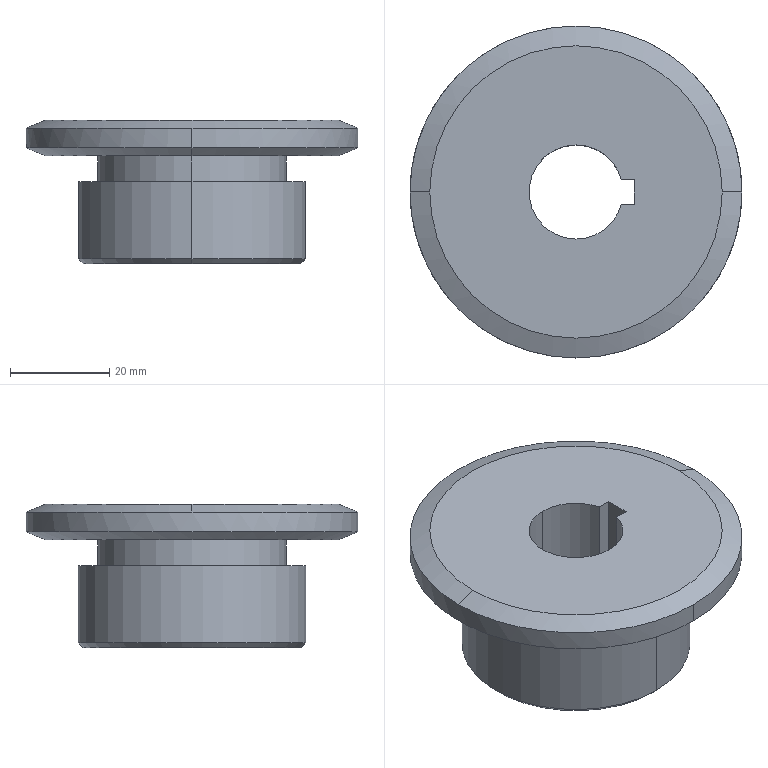Component | SolidWorks | YC1-250-03-01SliderAssembly-1_YC1-200-03-33SmallSprocket-1 | 1 solid | 23 faces | box 67 x 67 x 29 mm | volume 48926 mm3 | cylinder 9 | cone 7 | plane 7 | commonest cylinder face diameters 19 x3 67 x2 46 x2 38 x2 | material Plain Carbon Steel
STEP:
#1=COLOUR_RGB('',0.7922,0.8196,0.9333);
#2=FILL_AREA_STYLE_COLOUR('',#1);
#3=FILL_AREA_STYLE('',(#2));
#4=SURFACE_STYLE_FILL_AREA(#3);
#5=SURFACE_SIDE_STYLE('',(#4));
#6=SURFACE_STYLE_USAGE(.BOTH.,#5);
#7=PRESENTATION_STYLE_ASSIGNMENT((#6));
#8=CARTESIAN_POINT('',(8.248,68.998,-12.283));
#9=VERTEX_POINT('',#8);
#10=CARTESIAN_POINT('',(5.925,68.998,-12.283));
#11=VERTEX_POINT('',#10);
#12=CARTESIAN_POINT('',(7.087,68.998,-12.283));
#13=DIRECTION('',(0.,-0.,-1.));
#14=DIRECTION('',(1.,-0.,0.));
#15=AXIS2_PLACEMENT_3D('',#12,#13,#14);
#16=CIRCLE('',#15,1.161);
#17=EDGE_CURVE('',#9,#11,#16,.T.);
#18=ORIENTED_EDGE('',*,*,#17,.T.);
#19=CARTESIAN_POINT('',(5.768,68.998,-12.346));
#20=VERTEX_POINT('',#19);
#21=CARTESIAN_POINT('',(5.768,68.998,-12.346));
#22=DIRECTION('',(-0.9285,0.,-0.3714));
#23=VECTOR('',#22,39.37);
#24=LINE('',#21,#23);
#25=EDGE_CURVE('',#11,#20,#24,.T.);
#26=ORIENTED_EDGE('',*,*,#25,.T.);
#27=CARTESIAN_POINT('',(7.087,67.679,-12.346));
#28=VERTEX_POINT('',#27);
#29=CARTESIAN_POINT('',(7.087,68.998,-12.346));
#30=DIRECTION('',(0.,0.,1.));
#31=DIRECTION('',(0.,1.,0.));
#32=AXIS2_PLACEMENT_3D('',#29,#30,#31);
#33=CIRCLE('',#32,1.319);
#34=EDGE_CURVE('',#20,#28,#33,.T.);
#35=ORIENTED_EDGE('',*,*,#34,.T.);
#36=CARTESIAN_POINT('',(8.406,68.998,-12.346));
#37=VERTEX_POINT('',#36);
#38=CARTESIAN_POINT('',(7.087,68.998,-12.346));
#39=DIRECTION('',(0.,0.,1.));
#40=DIRECTION('',(0.,1.,0.));
#41=AXIS2_PLACEMENT_3D('',#38,#39,#40);
#42=CIRCLE('',#41,1.319);
#43=EDGE_CURVE('',#28,#37,#42,.T.);
#44=ORIENTED_EDGE('',*,*,#43,.T.);
#45=CARTESIAN_POINT('',(8.406,68.998,-12.346));
#46=DIRECTION('',(0.9285,-0.,-0.3714));
#47=VECTOR('',#46,39.37);
#48=LINE('',#45,#47);
#49=EDGE_CURVE('',#9,#37,#48,.T.);
#50=ORIENTED_EDGE('',*,*,#49,.F.);
#51=EDGE_LOOP('',(#18,#26,#35,#44,#50));
#52=FACE_OUTER_BOUND('',#51,.T.);
#53=CARTESIAN_POINT('',(7.087,68.998,-12.346));
#54=DIRECTION('',(0.,-0.,-1.));
#55=DIRECTION('',(1.,-0.,0.));
#56=AXIS2_PLACEMENT_3D('',#53,#54,#55);
#57=CONICAL_SURFACE('',#56,1.319,1.19);
#58=ADVANCED_FACE('',(#52),#57,.T.);
#59=CARTESIAN_POINT('',(7.087,69.372,-13.406));
#60=VERTEX_POINT('',#59);
#61=CARTESIAN_POINT('',(7.087,68.624,-13.406));
#62=VERTEX_POINT('',#61);
#63=CARTESIAN_POINT('',(7.087,68.998,-13.406));
#64=DIRECTION('',(0.,0.,1.));
#65=DIRECTION('',(-0.,-1.,0.));
#66=AXIS2_PLACEMENT_3D('',#63,#64,#65);
#67=CIRCLE('',#66,0.374);
#68=EDGE_CURVE('',#60,#62,#67,.T.);
#69=ORIENTED_EDGE('',*,*,#68,.F.);
#70=CARTESIAN_POINT('',(7.087,69.372,-12.283));
#71=VERTEX_POINT('',#70);
#72=CARTESIAN_POINT('',(7.087,69.372,-12.283));
#73=DIRECTION('',(0.,0.,1.));
#74=VECTOR('',#73,39.37);
#75=LINE('',#72,#74);
#76=EDGE_CURVE('',#60,#71,#75,.T.);
#77=ORIENTED_EDGE('',*,*,#76,.T.);
#78=CARTESIAN_POINT('',(7.087,68.624,-12.283));
#79=VERTEX_POINT('',#78);
#80=CARTESIAN_POINT('',(7.087,68.998,-12.283));
#81=DIRECTION('',(0.,0.,1.));
#82=DIRECTION('',(-0.,-1.,0.));
#83=AXIS2_PLACEMENT_3D('',#80,#81,#82);
#84=CIRCLE('',#83,0.374);
#85=EDGE_CURVE('',#71,#79,#84,.T.);
#86=ORIENTED_EDGE('',*,*,#85,.T.);
#87=CARTESIAN_POINT('',(7.087,68.624,-12.283));
#88=DIRECTION('',(0.,0.,1.));
#89=VECTOR('',#88,39.37);
#90=LINE('',#87,#89);
#91=EDGE_CURVE('',#62,#79,#90,.T.);
#92=ORIENTED_EDGE('',*,*,#91,.F.);
#93=EDGE_LOOP('',(#69,#77,#86,#92));
#94=FACE_OUTER_BOUND('',#93,.T.);
#95=CARTESIAN_POINT('',(7.087,68.998,-12.283));
#96=DIRECTION('',(0.,0.,1.));
#97=DIRECTION('',(-0.,-1.,0.));
#98=AXIS2_PLACEMENT_3D('',#95,#96,#97);
#99=CYLINDRICAL_SURFACE('',#98,0.374);
#100=ADVANCED_FACE('',(#94),#99,.F.);
#101=CARTESIAN_POINT('',(7.447,68.899,-13.406));
#102=VERTEX_POINT('',#101);
#103=CARTESIAN_POINT('',(7.087,68.998,-13.406));
#104=DIRECTION('',(0.,0.,1.));
#105=DIRECTION('',(-0.,-1.,0.));
#106=AXIS2_PLACEMENT_3D('',#103,#104,#105);
#107=CIRCLE('',#106,0.374);
#108=EDGE_CURVE('',#62,#102,#107,.T.);
#109=ORIENTED_EDGE('',*,*,#108,.F.);
#110=ORIENTED_EDGE('',*,*,#91,.T.);
#111=CARTESIAN_POINT('',(7.447,68.899,-12.283));
#112=VERTEX_POINT('',#111);
#113=CARTESIAN_POINT('',(7.087,68.998,-12.283));
#114=DIRECTION('',(0.,0.,1.));
#115=DIRECTION('',(-0.,-1.,0.));
#116=AXIS2_PLACEMENT_3D('',#113,#114,#115);
#117=CIRCLE('',#116,0.374);
#118=EDGE_CURVE('',#79,#112,#117,.T.);
#119=ORIENTED_EDGE('',*,*,#118,.T.);
#120=CARTESIAN_POINT('',(7.447,68.899,-12.283));
#121=DIRECTION('',(0.,0.,-1.));
#122=VECTOR('',#121,39.37);
#123=LINE('',#120,#122);
#124=EDGE_CURVE('',#112,#102,#123,.T.);
#125=ORIENTED_EDGE('',*,*,#124,.T.);
#126=EDGE_LOOP('',(#109,#110,#119,#125));
#127=FACE_OUTER_BOUND('',#126,.T.);
#128=CARTESIAN_POINT('',(7.087,68.998,-12.283));
#129=DIRECTION('',(0.,0.,1.));
#130=DIRECTION('',(-0.,-1.,0.));
#131=AXIS2_PLACEMENT_3D('',#128,#129,#130);
#132=CYLINDRICAL_SURFACE('',#131,0.374);
#133=ADVANCED_FACE('',(#127),#132,.F.);
#134=CARTESIAN_POINT('',(7.087,67.679,-12.504));
#135=VERTEX_POINT('',#134);
#136=CARTESIAN_POINT('',(7.087,70.317,-12.504));
#137=VERTEX_POINT('',#136);
#138=CARTESIAN_POINT('',(7.087,68.998,-12.504));
#139=DIRECTION('',(0.,0.,1.));
#140=DIRECTION('',(-0.,-1.,0.));
#141=AXIS2_PLACEMENT_3D('',#138,#139,#140);
#142=CIRCLE('',#141,1.319);
#143=EDGE_CURVE('',#135,#137,#142,.T.);
#144=ORIENTED_EDGE('',*,*,#143,.T.);
#145=CARTESIAN_POINT('',(7.087,70.317,-12.346));
#146=VERTEX_POINT('',#145);
#147=CARTESIAN_POINT('',(7.087,70.317,-12.283));
#148=DIRECTION('',(0.,0.,1.));
#149=VECTOR('',#148,39.37);
#150=LINE('',#147,#149);
#151=EDGE_CURVE('',#137,#146,#150,.T.);
#152=ORIENTED_EDGE('',*,*,#151,.T.);
#153=CARTESIAN_POINT('',(7.087,68.998,-12.346));
#154=DIRECTION('',(0.,0.,1.));
#155=DIRECTION('',(0.,1.,0.));
#156=AXIS2_PLACEMENT_3D('',#153,#154,#155);
#157=CIRCLE('',#156,1.319);
#158=EDGE_CURVE('',#37,#146,#157,.T.);
#159=ORIENTED_EDGE('',*,*,#158,.F.);
#160=ORIENTED_EDGE('',*,*,#43,.F.);
#161=CARTESIAN_POINT('',(7.087,67.679,-12.283));
#162=DIRECTION('',(0.,0.,1.));
#163=VECTOR('',#162,39.37);
#164=LINE('',#161,#163);
#165=EDGE_CURVE('',#135,#28,#164,.T.);
#166=ORIENTED_EDGE('',*,*,#165,.F.);
#167=EDGE_LOOP('',(#144,#152,#159,#160,#166));
#168=FACE_OUTER_BOUND('',#167,.T.);
#169=CARTESIAN_POINT('',(7.087,68.998,-12.283));
#170=DIRECTION('',(0.,0.,1.));
#171=DIRECTION('',(-0.,-1.,0.));
#172=AXIS2_PLACEMENT_3D('',#169,#170,#171);
#173=CYLINDRICAL_SURFACE('',#172,1.319);
#174=ADVANCED_FACE('',(#168),#173,.T.);
#175=CARTESIAN_POINT('',(7.087,67.836,-12.567));
#176=VERTEX_POINT('',#175);
#177=CARTESIAN_POINT('',(7.087,70.159,-12.567));
#178=VERTEX_POINT('',#177);
#179=CARTESIAN_POINT('',(7.087,68.998,-12.567));
#180=DIRECTION('',(0.,0.,1.));
#181=DIRECTION('',(-0.,-1.,0.));
#182=AXIS2_PLACEMENT_3D('',#179,#180,#181);
#183=CIRCLE('',#182,1.161);
#184=EDGE_CURVE('',#176,#178,#183,.T.);
#185=ORIENTED_EDGE('',*,*,#184,.T.);
#186=CARTESIAN_POINT('',(7.087,70.317,-12.504));
#187=DIRECTION('',(0.,0.9285,0.3714));
#188=VECTOR('',#187,39.37);
#189=LINE('',#186,#188);
#190=EDGE_CURVE('',#178,#137,#189,.T.);
#191=ORIENTED_EDGE('',*,*,#190,.T.);
#192=ORIENTED_EDGE('',*,*,#143,.F.);
#193=CARTESIAN_POINT('',(7.087,67.679,-12.504));
#194=DIRECTION('',(-0.,-0.9285,0.3714));
#195=VECTOR('',#194,39.37);
#196=LINE('',#193,#195);
#197=EDGE_CURVE('',#176,#135,#196,.T.);
#198=ORIENTED_EDGE('',*,*,#197,.F.);
#199=EDGE_LOOP('',(#185,#191,#192,#198));
#200=FACE_OUTER_BOUND('',#199,.T.);
#201=CARTESIAN_POINT('',(7.087,68.998,-12.504));
#202=DIRECTION('',(0.,0.,1.));
#203=DIRECTION('',(-0.,-1.,0.));
#204=AXIS2_PLACEMENT_3D('',#201,#202,#203);
#205=CONICAL_SURFACE('',#204,1.319,1.19);
#206=ADVANCED_FACE('',(#200),#205,.T.);
#207=CARTESIAN_POINT('',(7.087,68.132,-13.425));
#208=VERTEX_POINT('',#207);
#209=CARTESIAN_POINT('',(7.087,69.864,-13.425));
#210=VERTEX_POINT('',#209);
#211=CARTESIAN_POINT('',(7.087,68.998,-13.425));
#212=DIRECTION('',(0.,0.,1.));
#213=DIRECTION('',(-0.,-1.,0.));
#214=AXIS2_PLACEMENT_3D('',#211,#212,#213);
#215=CIRCLE('',#214,0.8661);
#216=EDGE_CURVE('',#208,#210,#215,.T.);
#217=ORIENTED_EDGE('',*,*,#216,.T.);
#218=CARTESIAN_POINT('',(7.087,69.903,-13.386));
#219=VERTEX_POINT('',#218);
#220=CARTESIAN_POINT('',(7.087,69.903,-13.386));
#221=DIRECTION('',(0.,0.7071,0.7071));
#222=VECTOR('',#221,39.37);
#223=LINE('',#220,#222);
#224=EDGE_CURVE('',#210,#219,#223,.T.);
#225=ORIENTED_EDGE('',*,*,#224,.T.);
#226=CARTESIAN_POINT('',(7.087,68.092,-13.386));
#227=VERTEX_POINT('',#226);
#228=CARTESIAN_POINT('',(7.087,68.998,-13.386));
#229=DIRECTION('',(0.,0.,-1.));
#230=DIRECTION('',(-0.,-1.,0.));
#231=AXIS2_PLACEMENT_3D('',#228,#229,#230);
#232=CIRCLE('',#231,0.9055);
#233=EDGE_CURVE('',#219,#227,#232,.T.);
#234=ORIENTED_EDGE('',*,*,#233,.T.);
#235=CARTESIAN_POINT('',(7.087,68.092,-13.386));
#236=DIRECTION('',(-0.,-0.7071,0.7071));
#237=VECTOR('',#236,39.37);
#238=LINE('',#235,#237);
#239=EDGE_CURVE('',#208,#227,#238,.T.);
#240=ORIENTED_EDGE('',*,*,#239,.F.);
#241=EDGE_LOOP('',(#217,#225,#234,#240));
#242=FACE_OUTER_BOUND('',#241,.T.);
#243=CARTESIAN_POINT('',(7.087,68.998,-13.386));
#244=DIRECTION('',(0.,0.,1.));
#245=DIRECTION('',(-0.,-1.,0.));
#246=AXIS2_PLACEMENT_3D('',#243,#244,#245);
#247=CONICAL_SURFACE('',#246,0.9055,0.7854);
#248=ADVANCED_FACE('',(#242),#247,.T.);
#249=ORIENTED_EDGE('',*,*,#233,.F.);
#250=CARTESIAN_POINT('',(7.087,69.903,-12.772));
#251=VERTEX_POINT('',#250);
#252=CARTESIAN_POINT('',(7.087,69.903,-12.283));
#253=DIRECTION('',(0.,0.,1.));
#254=VECTOR('',#253,39.37);
#255=LINE('',#252,#254);
#256=EDGE_CURVE('',#219,#251,#255,.T.);
#257=ORIENTED_EDGE('',*,*,#256,.T.);
#258=CARTESIAN_POINT('',(7.087,68.092,-12.772));
#259=VERTEX_POINT('',#258);
#260=CARTESIAN_POINT('',(7.087,68.998,-12.772));
#261=DIRECTION('',(0.,0.,-1.));
#262=DIRECTION('',(-0.,-1.,0.));
#263=AXIS2_PLACEMENT_3D('',#260,#261,#262);
#264=CIRCLE('',#263,0.9055);
#265=EDGE_CURVE('',#251,#259,#264,.T.);
#266=ORIENTED_EDGE('',*,*,#265,.T.);
#267=CARTESIAN_POINT('',(7.087,68.092,-12.283));
#268=DIRECTION('',(0.,0.,1.));
#269=VECTOR('',#268,39.37);
#270=LINE('',#267,#269);
#271=EDGE_CURVE('',#227,#259,#270,.T.);
#272=ORIENTED_EDGE('',*,*,#271,.F.);
#273=EDGE_LOOP('',(#249,#257,#266,#272));
#274=FACE_OUTER_BOUND('',#273,.T.);
#275=CARTESIAN_POINT('',(7.087,68.998,-12.283));
#276=DIRECTION('',(0.,0.,1.));
#277=DIRECTION('',(-0.,-1.,0.));
#278=AXIS2_PLACEMENT_3D('',#275,#276,#277);
#279=CYLINDRICAL_SURFACE('',#278,0.9055);
#280=ADVANCED_FACE('',(#274),#279,.T.);
#281=CARTESIAN_POINT('',(7.087,68.25,-12.772));
#282=VERTEX_POINT('',#281);
#283=CARTESIAN_POINT('',(7.087,69.746,-12.772));
#284=VERTEX_POINT('',#283);
#285=CARTESIAN_POINT('',(7.087,68.998,-12.772));
#286=DIRECTION('',(0.,0.,1.));
#287=DIRECTION('',(-0.,-1.,0.));
#288=AXIS2_PLACEMENT_3D('',#285,#286,#287);
#289=CIRCLE('',#288,0.748);
#290=EDGE_CURVE('',#282,#284,#289,.T.);
#291=ORIENTED_EDGE('',*,*,#290,.T.);
#292=CARTESIAN_POINT('',(7.087,69.746,-12.567));
#293=VERTEX_POINT('',#292);
#294=CARTESIAN_POINT('',(7.087,69.746,-12.283));
#295=DIRECTION('',(0.,0.,1.));
#296=VECTOR('',#295,39.37);
#297=LINE('',#294,#296);
#298=EDGE_CURVE('',#284,#293,#297,.T.);
#299=ORIENTED_EDGE('',*,*,#298,.T.);
#300=CARTESIAN_POINT('',(7.087,68.25,-12.567));
#301=VERTEX_POINT('',#300);
#302=CARTESIAN_POINT('',(7.087,68.998,-12.567));
#303=DIRECTION('',(0.,0.,-1.));
#304=DIRECTION('',(-0.,-1.,0.));
#305=AXIS2_PLACEMENT_3D('',#302,#303,#304);
#306=CIRCLE('',#305,0.748);
#307=EDGE_CURVE('',#293,#301,#306,.T.);
#308=ORIENTED_EDGE('',*,*,#307,.T.);
#309=CARTESIAN_POINT('',(7.087,68.25,-12.283));
#310=DIRECTION('',(0.,0.,1.));
#311=VECTOR('',#310,39.37);
#312=LINE('',#309,#311);
#313=EDGE_CURVE('',#282,#301,#312,.T.);
#314=ORIENTED_EDGE('',*,*,#313,.F.);
#315=EDGE_LOOP('',(#291,#299,#308,#314));
#316=FACE_OUTER_BOUND('',#315,.T.);
#317=CARTESIAN_POINT('',(7.087,68.998,-12.283));
#318=DIRECTION('',(0.,0.,1.));
#319=DIRECTION('',(-0.,-1.,0.));
#320=AXIS2_PLACEMENT_3D('',#317,#318,#319);
#321=CYLINDRICAL_SURFACE('',#320,0.748);
#322=ADVANCED_FACE('',(#316),#321,.T.);
#323=ORIENTED_EDGE('',*,*,#17,.F.);
#324=CARTESIAN_POINT('',(7.087,68.998,-12.283));
#325=DIRECTION('',(0.,-0.,-1.));
#326=DIRECTION('',(1.,-0.,0.));
#327=AXIS2_PLACEMENT_3D('',#324,#325,#326);
#328=CIRCLE('',#327,1.161);
#329=EDGE_CURVE('',#11,#9,#328,.T.);
#330=ORIENTED_EDGE('',*,*,#329,.F.);
#331=EDGE_LOOP('',(#323,#330));
#332=FACE_OUTER_BOUND('',#331,.T.);
#333=CARTESIAN_POINT('',(7.551,69.096,-12.283));
#334=VERTEX_POINT('',#333);
#335=CARTESIAN_POINT('',(7.447,69.096,-12.283));
#336=VERTEX_POINT('',#335);
#337=CARTESIAN_POINT('',(8.248,69.096,-12.283));
#338=DIRECTION('',(-1.,0.,0.));
#339=VECTOR('',#338,39.37);
#340=LINE('',#337,#339);
#341=EDGE_CURVE('',#334,#336,#340,.T.);
#342=ORIENTED_EDGE('',*,*,#341,.F.);
#343=CARTESIAN_POINT('',(7.551,68.899,-12.283));
#344=VERTEX_POINT('',#343);
#345=CARTESIAN_POINT('',(7.551,68.998,-12.283));
#346=DIRECTION('',(0.,1.,0.));
#347=VECTOR('',#346,39.37);
#348=LINE('',#345,#347);
#349=EDGE_CURVE('',#344,#334,#348,.T.);
#350=ORIENTED_EDGE('',*,*,#349,.F.);
#351=CARTESIAN_POINT('',(8.248,68.899,-12.283));
#352=DIRECTION('',(1.,-0.,0.));
#353=VECTOR('',#352,39.37);
#354=LINE('',#351,#353);
#355=EDGE_CURVE('',#112,#344,#354,.T.);
#356=ORIENTED_EDGE('',*,*,#355,.F.);
#357=ORIENTED_EDGE('',*,*,#118,.F.);
#358=ORIENTED_EDGE('',*,*,#85,.F.);
#359=CARTESIAN_POINT('',(7.087,68.998,-12.283));
#360=DIRECTION('',(0.,0.,1.));
#361=DIRECTION('',(-0.,-1.,0.));
#362=AXIS2_PLACEMENT_3D('',#359,#360,#361);
#363=CIRCLE('',#362,0.374);
#364=EDGE_CURVE('',#336,#71,#363,.T.);
#365=ORIENTED_EDGE('',*,*,#364,.F.);
#366=EDGE_LOOP('',(#342,#350,#356,#357,#358,#365));
#367=FACE_BOUND('',#366,.T.);
#368=CARTESIAN_POINT('',(8.248,68.998,-12.283));
#369=DIRECTION('',(0.,0.,-1.));
#370=DIRECTION('',(0.,1.,0.));
#371=AXIS2_PLACEMENT_3D('',#368,#369,#370);
#372=PLANE('',#371);
#373=ADVANCED_FACE('',(#332,#367),#372,.F.);
#374=ORIENTED_EDGE('',*,*,#25,.F.);
#375=ORIENTED_EDGE('',*,*,#329,.T.);
#376=ORIENTED_EDGE('',*,*,#49,.T.);
#377=ORIENTED_EDGE('',*,*,#158,.T.);
#378=CARTESIAN_POINT('',(7.087,68.998,-12.346));
#379=DIRECTION('',(0.,0.,1.));
#380=DIRECTION('',(0.,1.,0.));
#381=AXIS2_PLACEMENT_3D('',#378,#379,#380);
#382=CIRCLE('',#381,1.319);
#383=EDGE_CURVE('',#146,#20,#382,.T.);
#384=ORIENTED_EDGE('',*,*,#383,.T.);
#385=EDGE_LOOP('',(#374,#375,#376,#377,#384));
#386=FACE_OUTER_BOUND('',#385,.T.);
#387=CARTESIAN_POINT('',(7.087,68.998,-12.346));
#388=DIRECTION('',(0.,-0.,-1.));
#389=DIRECTION('',(1.,-0.,0.));
#390=AXIS2_PLACEMENT_3D('',#387,#388,#389);
#391=CONICAL_SURFACE('',#390,1.319,1.19);
#392=ADVANCED_FACE('',(#386),#391,.T.);
#393=ORIENTED_EDGE('',*,*,#76,.F.);
#394=CARTESIAN_POINT('',(7.447,69.096,-13.406));
#395=VERTEX_POINT('',#394);
#396=CARTESIAN_POINT('',(7.087,68.998,-13.406));
#397=DIRECTION('',(0.,0.,1.));
#398=DIRECTION('',(-0.,-1.,0.));
#399=AXIS2_PLACEMENT_3D('',#396,#397,#398);
#400=CIRCLE('',#399,0.374);
#401=EDGE_CURVE('',#395,#60,#400,.T.);
#402=ORIENTED_EDGE('',*,*,#401,.F.);
#403=CARTESIAN_POINT('',(7.447,69.096,-12.283));
#404=DIRECTION('',(0.,0.,-1.));
#405=VECTOR('',#404,39.37);
#406=LINE('',#403,#405);
#407=EDGE_CURVE('',#336,#395,#406,.T.);
#408=ORIENTED_EDGE('',*,*,#407,.F.);
#409=ORIENTED_EDGE('',*,*,#364,.T.);
#410=EDGE_LOOP('',(#393,#402,#408,#409));
#411=FACE_OUTER_BOUND('',#410,.T.);
#412=CARTESIAN_POINT('',(7.087,68.998,-12.283));
#413=DIRECTION('',(0.,0.,1.));
#414=DIRECTION('',(-0.,-1.,0.));
#415=AXIS2_PLACEMENT_3D('',#412,#413,#414);
#416=CYLINDRICAL_SURFACE('',#415,0.374);
#417=ADVANCED_FACE('',(#411),#416,.F.);
#418=CARTESIAN_POINT('',(7.468,69.096,-13.425));
#419=VERTEX_POINT('',#418);
#420=CARTESIAN_POINT('',(7.468,69.096,-13.425));
#421=CARTESIAN_POINT('',(7.461,69.096,-13.419));
#422=CARTESIAN_POINT('',(7.454,69.096,-13.412));
#423=CARTESIAN_POINT('',(7.447,69.096,-13.406));
#424=B_SPLINE_CURVE_WITH_KNOTS('',3,(#420,#421,#422,#423),.UNSPECIFIED.,.F.,.F.,(4,4),(0.,0.0007194),.UNSPECIFIED.);
#425=EDGE_CURVE('',#419,#395,#424,.T.);
#426=ORIENTED_EDGE('',*,*,#425,.F.);
#427=CARTESIAN_POINT('',(7.551,69.096,-13.425));
#428=VERTEX_POINT('',#427);
#429=CARTESIAN_POINT('',(7.447,69.096,-13.425));
#430=DIRECTION('',(-1.,0.,0.));
#431=VECTOR('',#430,39.37);
#432=LINE('',#429,#431);
#433=EDGE_CURVE('',#428,#419,#432,.T.);
#434=ORIENTED_EDGE('',*,*,#433,.F.);
#435=CARTESIAN_POINT('',(7.551,69.096,-12.283));
#436=DIRECTION('',(0.,0.,-1.));
#437=VECTOR('',#436,39.37);
#438=LINE('',#435,#437);
#439=EDGE_CURVE('',#334,#428,#438,.T.);
#440=ORIENTED_EDGE('',*,*,#439,.F.);
#441=ORIENTED_EDGE('',*,*,#341,.T.);
#442=ORIENTED_EDGE('',*,*,#407,.T.);
#443=EDGE_LOOP('',(#426,#434,#440,#441,#442));
#444=FACE_OUTER_BOUND('',#443,.T.);
#445=CARTESIAN_POINT('',(7.447,69.096,-12.283));
#446=DIRECTION('',(0.,1.,0.));
#447=DIRECTION('',(0.,0.,1.));
#448=AXIS2_PLACEMENT_3D('',#445,#446,#447);
#449=PLANE('',#448);
#450=ADVANCED_FACE('',(#444),#449,.F.);
#451=CARTESIAN_POINT('',(7.551,68.899,-13.425));
#452=VERTEX_POINT('',#451);
#453=CARTESIAN_POINT('',(7.551,68.899,-12.283));
#454=DIRECTION('',(0.,0.,-1.));
#455=VECTOR('',#454,39.37);
#456=LINE('',#453,#455);
#457=EDGE_CURVE('',#344,#452,#456,.T.);
#458=ORIENTED_EDGE('',*,*,#457,.F.);
#459=ORIENTED_EDGE('',*,*,#349,.T.);
#460=ORIENTED_EDGE('',*,*,#439,.T.);
#461=CARTESIAN_POINT('',(7.551,68.899,-13.425));
#462=DIRECTION('',(0.,1.,0.));
#463=VECTOR('',#462,39.37);
#464=LINE('',#461,#463);
#465=EDGE_CURVE('',#452,#428,#464,.T.);
#466=ORIENTED_EDGE('',*,*,#465,.F.);
#467=EDGE_LOOP('',(#458,#459,#460,#466));
#468=FACE_OUTER_BOUND('',#467,.T.);
#469=CARTESIAN_POINT('',(7.551,68.899,-12.283));
#470=DIRECTION('',(1.,-0.,0.));
#471=DIRECTION('',(0.,0.,1.));
#472=AXIS2_PLACEMENT_3D('',#469,#470,#471);
#473=PLANE('',#472);
#474=ADVANCED_FACE('',(#468),#473,.F.);
#475=CARTESIAN_POINT('',(7.468,68.899,-13.425));
#476=VERTEX_POINT('',#475);
#477=CARTESIAN_POINT('',(7.468,68.899,-13.425));
#478=CARTESIAN_POINT('',(7.461,68.899,-13.419));
#479=CARTESIAN_POINT('',(7.454,68.899,-13.412));
#480=CARTESIAN_POINT('',(7.447,68.899,-13.406));
#481=B_SPLINE_CURVE_WITH_KNOTS('',3,(#477,#478,#479,#480),.UNSPECIFIED.,.F.,.F.,(4,4),(0.,0.0007194),.UNSPECIFIED.);
#482=EDGE_CURVE('',#476,#102,#481,.T.);
#483=ORIENTED_EDGE('',*,*,#482,.T.);
#484=ORIENTED_EDGE('',*,*,#124,.F.);
#485=ORIENTED_EDGE('',*,*,#355,.T.);
#486=ORIENTED_EDGE('',*,*,#457,.T.);
#487=CARTESIAN_POINT('',(7.447,68.899,-13.425));
#488=DIRECTION('',(1.,-0.,0.));
#489=VECTOR('',#488,39.37);
#490=LINE('',#487,#489);
#491=EDGE_CURVE('',#476,#452,#490,.T.);
#492=ORIENTED_EDGE('',*,*,#491,.F.);
#493=EDGE_LOOP('',(#483,#484,#485,#486,#492));
#494=FACE_OUTER_BOUND('',#493,.T.);
#495=CARTESIAN_POINT('',(7.447,68.899,-12.283));
#496=DIRECTION('',(-0.,-1.,0.));
#497=DIRECTION('',(0.,0.,-1.));
#498=AXIS2_PLACEMENT_3D('',#495,#496,#497);
#499=PLANE('',#498);
#500=ADVANCED_FACE('',(#494),#499,.F.);
#501=ORIENTED_EDGE('',*,*,#151,.F.);
#502=CARTESIAN_POINT('',(7.087,68.998,-12.504));
#503=DIRECTION('',(0.,0.,1.));
#504=DIRECTION('',(-0.,-1.,0.));
#505=AXIS2_PLACEMENT_3D('',#502,#503,#504);
#506=CIRCLE('',#505,1.319);
#507=EDGE_CURVE('',#137,#135,#506,.T.);
#508=ORIENTED_EDGE('',*,*,#507,.T.);
#509=ORIENTED_EDGE('',*,*,#165,.T.);
#510=ORIENTED_EDGE('',*,*,#34,.F.);
#511=ORIENTED_EDGE('',*,*,#383,.F.);
#512=EDGE_LOOP('',(#501,#508,#509,#510,#511));
#513=FACE_OUTER_BOUND('',#512,.T.);
#514=CARTESIAN_POINT('',(7.087,68.998,-12.283));
#515=DIRECTION('',(0.,0.,1.));
#516=DIRECTION('',(-0.,-1.,0.));
#517=AXIS2_PLACEMENT_3D('',#514,#515,#516);
#518=CYLINDRICAL_SURFACE('',#517,1.319);
#519=ADVANCED_FACE('',(#513),#518,.T.);
#520=ORIENTED_EDGE('',*,*,#401,.T.);
#521=ORIENTED_EDGE('',*,*,#68,.T.);
#522=ORIENTED_EDGE('',*,*,#108,.T.);
#523=ORIENTED_EDGE('',*,*,#482,.F.);
#524=CARTESIAN_POINT('',(7.087,68.998,-13.425));
#525=DIRECTION('',(-0.,0.,1.));
#526=DIRECTION('',(1.,0.,0.));
#527=AXIS2_PLACEMENT_3D('',#524,#525,#526);
#528=CIRCLE('',#527,0.3937);
#529=EDGE_CURVE('',#419,#476,#528,.T.);
#530=ORIENTED_EDGE('',*,*,#529,.F.);
#531=ORIENTED_EDGE('',*,*,#425,.T.);
#532=EDGE_LOOP('',(#520,#521,#522,#523,#530,#531));
#533=FACE_OUTER_BOUND('',#532,.T.);
#534=CARTESIAN_POINT('',(7.087,68.998,-13.425));
#535=DIRECTION('',(0.,-0.,-1.));
#536=DIRECTION('',(1.,0.,0.));
#537=AXIS2_PLACEMENT_3D('',#534,#535,#536);
#538=CONICAL_SURFACE('',#537,0.3937,0.7854);
#539=ADVANCED_FACE('',(#533),#538,.F.);
#540=ORIENTED_EDGE('',*,*,#529,.T.);
#541=ORIENTED_EDGE('',*,*,#491,.T.);
#542=ORIENTED_EDGE('',*,*,#465,.T.);
#543=ORIENTED_EDGE('',*,*,#433,.T.);
#544=EDGE_LOOP('',(#540,#541,#542,#543));
#545=FACE_BOUND('',#544,.T.);
#546=ORIENTED_EDGE('',*,*,#216,.F.);
#547=CARTESIAN_POINT('',(7.087,68.998,-13.425));
#548=DIRECTION('',(0.,0.,1.));
#549=DIRECTION('',(-0.,-1.,0.));
#550=AXIS2_PLACEMENT_3D('',#547,#548,#549);
#551=CIRCLE('',#550,0.8661);
#552=EDGE_CURVE('',#210,#208,#551,.T.);
#553=ORIENTED_EDGE('',*,*,#552,.F.);
#554=EDGE_LOOP('',(#546,#553));
#555=FACE_OUTER_BOUND('',#554,.T.);
#556=CARTESIAN_POINT('',(7.461,68.998,-13.425));
#557=DIRECTION('',(0.,0.,1.));
#558=DIRECTION('',(-0.,-1.,0.));
#559=AXIS2_PLACEMENT_3D('',#556,#557,#558);
#560=PLANE('',#559);
#561=ADVANCED_FACE('',(#545,#555),#560,.F.);
#562=ORIENTED_EDGE('',*,*,#190,.F.);
#563=CARTESIAN_POINT('',(7.087,68.998,-12.567));
#564=DIRECTION('',(0.,0.,1.));
#565=DIRECTION('',(-0.,-1.,0.));
#566=AXIS2_PLACEMENT_3D('',#563,#564,#565);
#567=CIRCLE('',#566,1.161);
#568=EDGE_CURVE('',#178,#176,#567,.T.);
#569=ORIENTED_EDGE('',*,*,#568,.T.);
#570=ORIENTED_EDGE('',*,*,#197,.T.);
#571=ORIENTED_EDGE('',*,*,#507,.F.);
#572=EDGE_LOOP('',(#562,#569,#570,#571));
#573=FACE_OUTER_BOUND('',#572,.T.);
#574=CARTESIAN_POINT('',(7.087,68.998,-12.504));
#575=DIRECTION('',(0.,0.,1.));
#576=DIRECTION('',(-0.,-1.,0.));
#577=AXIS2_PLACEMENT_3D('',#574,#575,#576);
#578=CONICAL_SURFACE('',#577,1.319,1.19);
#579=ADVANCED_FACE('',(#573),#578,.T.);
#580=ORIENTED_EDGE('',*,*,#224,.F.);
#581=ORIENTED_EDGE('',*,*,#552,.T.);
#582=ORIENTED_EDGE('',*,*,#239,.T.);
#583=CARTESIAN_POINT('',(7.087,68.998,-13.386));
#584=DIRECTION('',(0.,0.,-1.));
#585=DIRECTION('',(-0.,-1.,0.));
#586=AXIS2_PLACEMENT_3D('',#583,#584,#585);
#587=CIRCLE('',#586,0.9055);
#588=EDGE_CURVE('',#227,#219,#587,.T.);
#589=ORIENTED_EDGE('',*,*,#588,.T.);
#590=EDGE_LOOP('',(#580,#581,#582,#589));
#591=FACE_OUTER_BOUND('',#590,.T.);
#592=CARTESIAN_POINT('',(7.087,68.998,-13.386));
#593=DIRECTION('',(0.,0.,1.));
#594=DIRECTION('',(-0.,-1.,0.));
#595=AXIS2_PLACEMENT_3D('',#592,#593,#594);
#596=CONICAL_SURFACE('',#595,0.9055,0.7854);
#597=ADVANCED_FACE('',(#591),#596,.T.);
#598=CARTESIAN_POINT('',(7.087,68.998,-12.567));
#599=DIRECTION('',(0.,0.,-1.));
#600=DIRECTION('',(-0.,-1.,0.));
#601=AXIS2_PLACEMENT_3D('',#598,#599,#600);
#602=CIRCLE('',#601,0.748);
#603=EDGE_CURVE('',#301,#293,#602,.T.);
#604=ORIENTED_EDGE('',*,*,#603,.F.);
#605=ORIENTED_EDGE('',*,*,#307,.F.);
#606=EDGE_LOOP('',(#604,#605));
#607=FACE_BOUND('',#606,.T.);
#608=ORIENTED_EDGE('',*,*,#184,.F.);
#609=ORIENTED_EDGE('',*,*,#568,.F.);
#610=EDGE_LOOP('',(#608,#609));
#611=FACE_OUTER_BOUND('',#610,.T.);
#612=CARTESIAN_POINT('',(7.835,68.998,-12.567));
#613=DIRECTION('',(0.,0.,1.));
#614=DIRECTION('',(-0.,-1.,0.));
#615=AXIS2_PLACEMENT_3D('',#612,#613,#614);
#616=PLANE('',#615);
#617=ADVANCED_FACE('',(#607,#611),#616,.F.);
#618=ORIENTED_EDGE('',*,*,#256,.F.);
#619=ORIENTED_EDGE('',*,*,#588,.F.);
#620=ORIENTED_EDGE('',*,*,#271,.T.);
#621=CARTESIAN_POINT('',(7.087,68.998,-12.772));
#622=DIRECTION('',(0.,0.,-1.));
#623=DIRECTION('',(-0.,-1.,0.));
#624=AXIS2_PLACEMENT_3D('',#621,#622,#623);
#625=CIRCLE('',#624,0.9055);
#626=EDGE_CURVE('',#259,#251,#625,.T.);
#627=ORIENTED_EDGE('',*,*,#626,.T.);
#628=EDGE_LOOP('',(#618,#619,#620,#627));
#629=FACE_OUTER_BOUND('',#628,.T.);
#630=CARTESIAN_POINT('',(7.087,68.998,-12.283));
#631=DIRECTION('',(0.,0.,1.));
#632=DIRECTION('',(-0.,-1.,0.));
#633=AXIS2_PLACEMENT_3D('',#630,#631,#632);
#634=CYLINDRICAL_SURFACE('',#633,0.9055);
#635=ADVANCED_FACE('',(#629),#634,.T.);
#636=ORIENTED_EDGE('',*,*,#298,.F.);
#637=CARTESIAN_POINT('',(7.087,68.998,-12.772));
#638=DIRECTION('',(0.,0.,1.));
#639=DIRECTION('',(-0.,-1.,0.));
#640=AXIS2_PLACEMENT_3D('',#637,#638,#639);
#641=CIRCLE('',#640,0.748);
#642=EDGE_CURVE('',#284,#282,#641,.T.);
#643=ORIENTED_EDGE('',*,*,#642,.T.);
#644=ORIENTED_EDGE('',*,*,#313,.T.);
#645=ORIENTED_EDGE('',*,*,#603,.T.);
#646=EDGE_LOOP('',(#636,#643,#644,#645));
#647=FACE_OUTER_BOUND('',#646,.T.);
#648=CARTESIAN_POINT('',(7.087,68.998,-12.283));
#649=DIRECTION('',(0.,0.,1.));
#650=DIRECTION('',(-0.,-1.,0.));
#651=AXIS2_PLACEMENT_3D('',#648,#649,#650);
#652=CYLINDRICAL_SURFACE('',#651,0.748);
#653=ADVANCED_FACE('',(#647),#652,.T.);
#654=ORIENTED_EDGE('',*,*,#626,.F.);
#655=ORIENTED_EDGE('',*,*,#265,.F.);
#656=EDGE_LOOP('',(#654,#655));
#657=FACE_OUTER_BOUND('',#656,.T.);
#658=ORIENTED_EDGE('',*,*,#290,.F.);
#659=ORIENTED_EDGE('',*,*,#642,.F.);
#660=EDGE_LOOP('',(#658,#659));
#661=FACE_BOUND('',#660,.T.);
#662=CARTESIAN_POINT('',(7.992,68.998,-12.772));
#663=DIRECTION('',(0.,0.,-1.));
#664=DIRECTION('',(0.,1.,0.));
#665=AXIS2_PLACEMENT_3D('',#662,#663,#664);
#666=PLANE('',#665);
#667=ADVANCED_FACE('',(#657,#661),#666,.F.);
#668=CLOSED_SHELL('',(#58,#100,#133,#174,#206,#248,#280,#322,#373,#392,#417,#450,#474,#500,#519,#539,#561,#579,#597,#617,#635,#653,#667));
#669=MANIFOLD_SOLID_BREP('',#668);
#670=STYLED_ITEM('',(#7),#669);
#671=(LENGTH_UNIT()NAMED_UNIT(*)SI_UNIT($,.METRE.));
#672=LENGTH_MEASURE_WITH_UNIT(LENGTH_MEASURE(0.0254),#671);
#673=DIMENSIONAL_EXPONENTS(1.,0.,0.,0.,0.,0.,0.);
#674=(CONVERSION_BASED_UNIT('',#672)LENGTH_UNIT()NAMED_UNIT(#673));
#675=UNCERTAINTY_MEASURE_WITH_UNIT(LENGTH_MEASURE(0.00001),#674,'','');
#676=(NAMED_UNIT(*)PLANE_ANGLE_UNIT()SI_UNIT($,.RADIAN.));
#677=(NAMED_UNIT(*)SI_UNIT($,.STERADIAN.)SOLID_ANGLE_UNIT());
#678=(GEOMETRIC_REPRESENTATION_CONTEXT(3)GLOBAL_UNCERTAINTY_ASSIGNED_CONTEXT((#675))GLOBAL_UNIT_ASSIGNED_CONTEXT((#674,#676,#677))REPRESENTATION_CONTEXT('',''));
#679=MECHANICAL_DESIGN_GEOMETRIC_PRESENTATION_REPRESENTATION('',(#670),#678);
#680=PRESENTATION_LAYER_ASSIGNMENT('','',(#670));
#681=CARTESIAN_POINT('',(0.,0.,0.));
#682=DIRECTION('',(0.,0.,1.));
#683=DIRECTION('',(1.,0.,0.));
#684=AXIS2_PLACEMENT_3D('',#681,#682,#683);
#685=(LENGTH_UNIT()NAMED_UNIT(*)SI_UNIT($,.METRE.));
#686=LENGTH_MEASURE_WITH_UNIT(LENGTH_MEASURE(0.0254),#685);
#687=DIMENSIONAL_EXPONENTS(1.,0.,0.,0.,0.,0.,0.);
#688=(CONVERSION_BASED_UNIT('',#686)LENGTH_UNIT()NAMED_UNIT(#687));
#689=UNCERTAINTY_MEASURE_WITH_UNIT(LENGTH_MEASURE(0.00001),#688,'','');
#690=(NAMED_UNIT(*)PLANE_ANGLE_UNIT()SI_UNIT($,.RADIAN.));
#691=(NAMED_UNIT(*)SI_UNIT($,.STERADIAN.)SOLID_ANGLE_UNIT());
#692=(GEOMETRIC_REPRESENTATION_CONTEXT(3)GLOBAL_UNCERTAINTY_ASSIGNED_CONTEXT((#689))GLOBAL_UNIT_ASSIGNED_CONTEXT((#688,#690,#691))REPRESENTATION_CONTEXT('',''));
#693=ADVANCED_BREP_SHAPE_REPRESENTATION('',(#669,#684),#692);